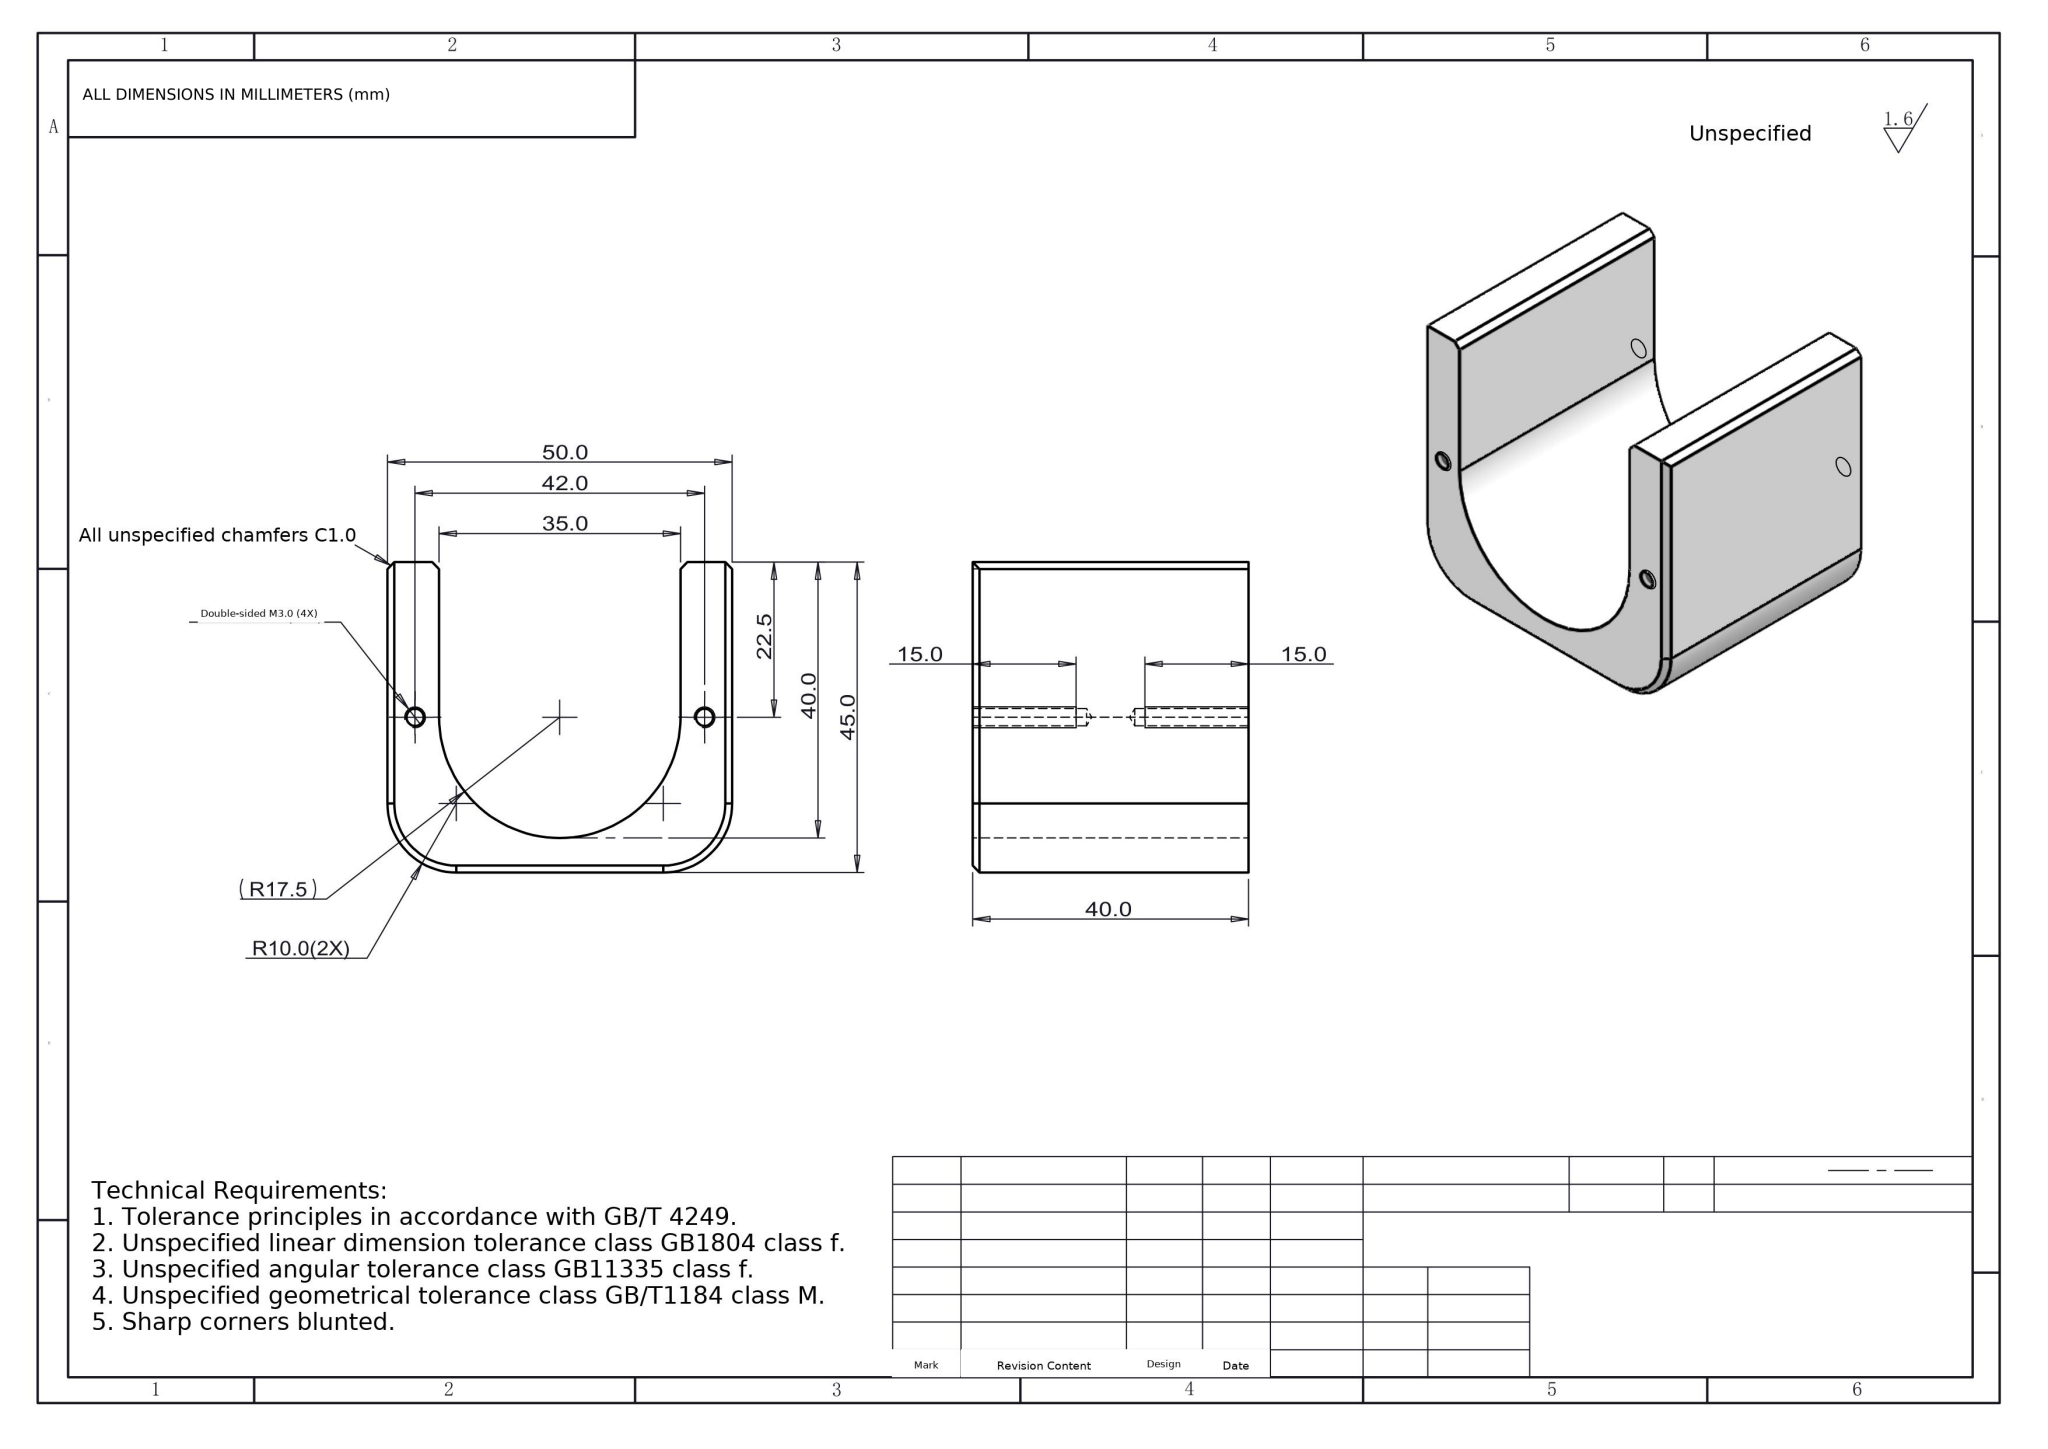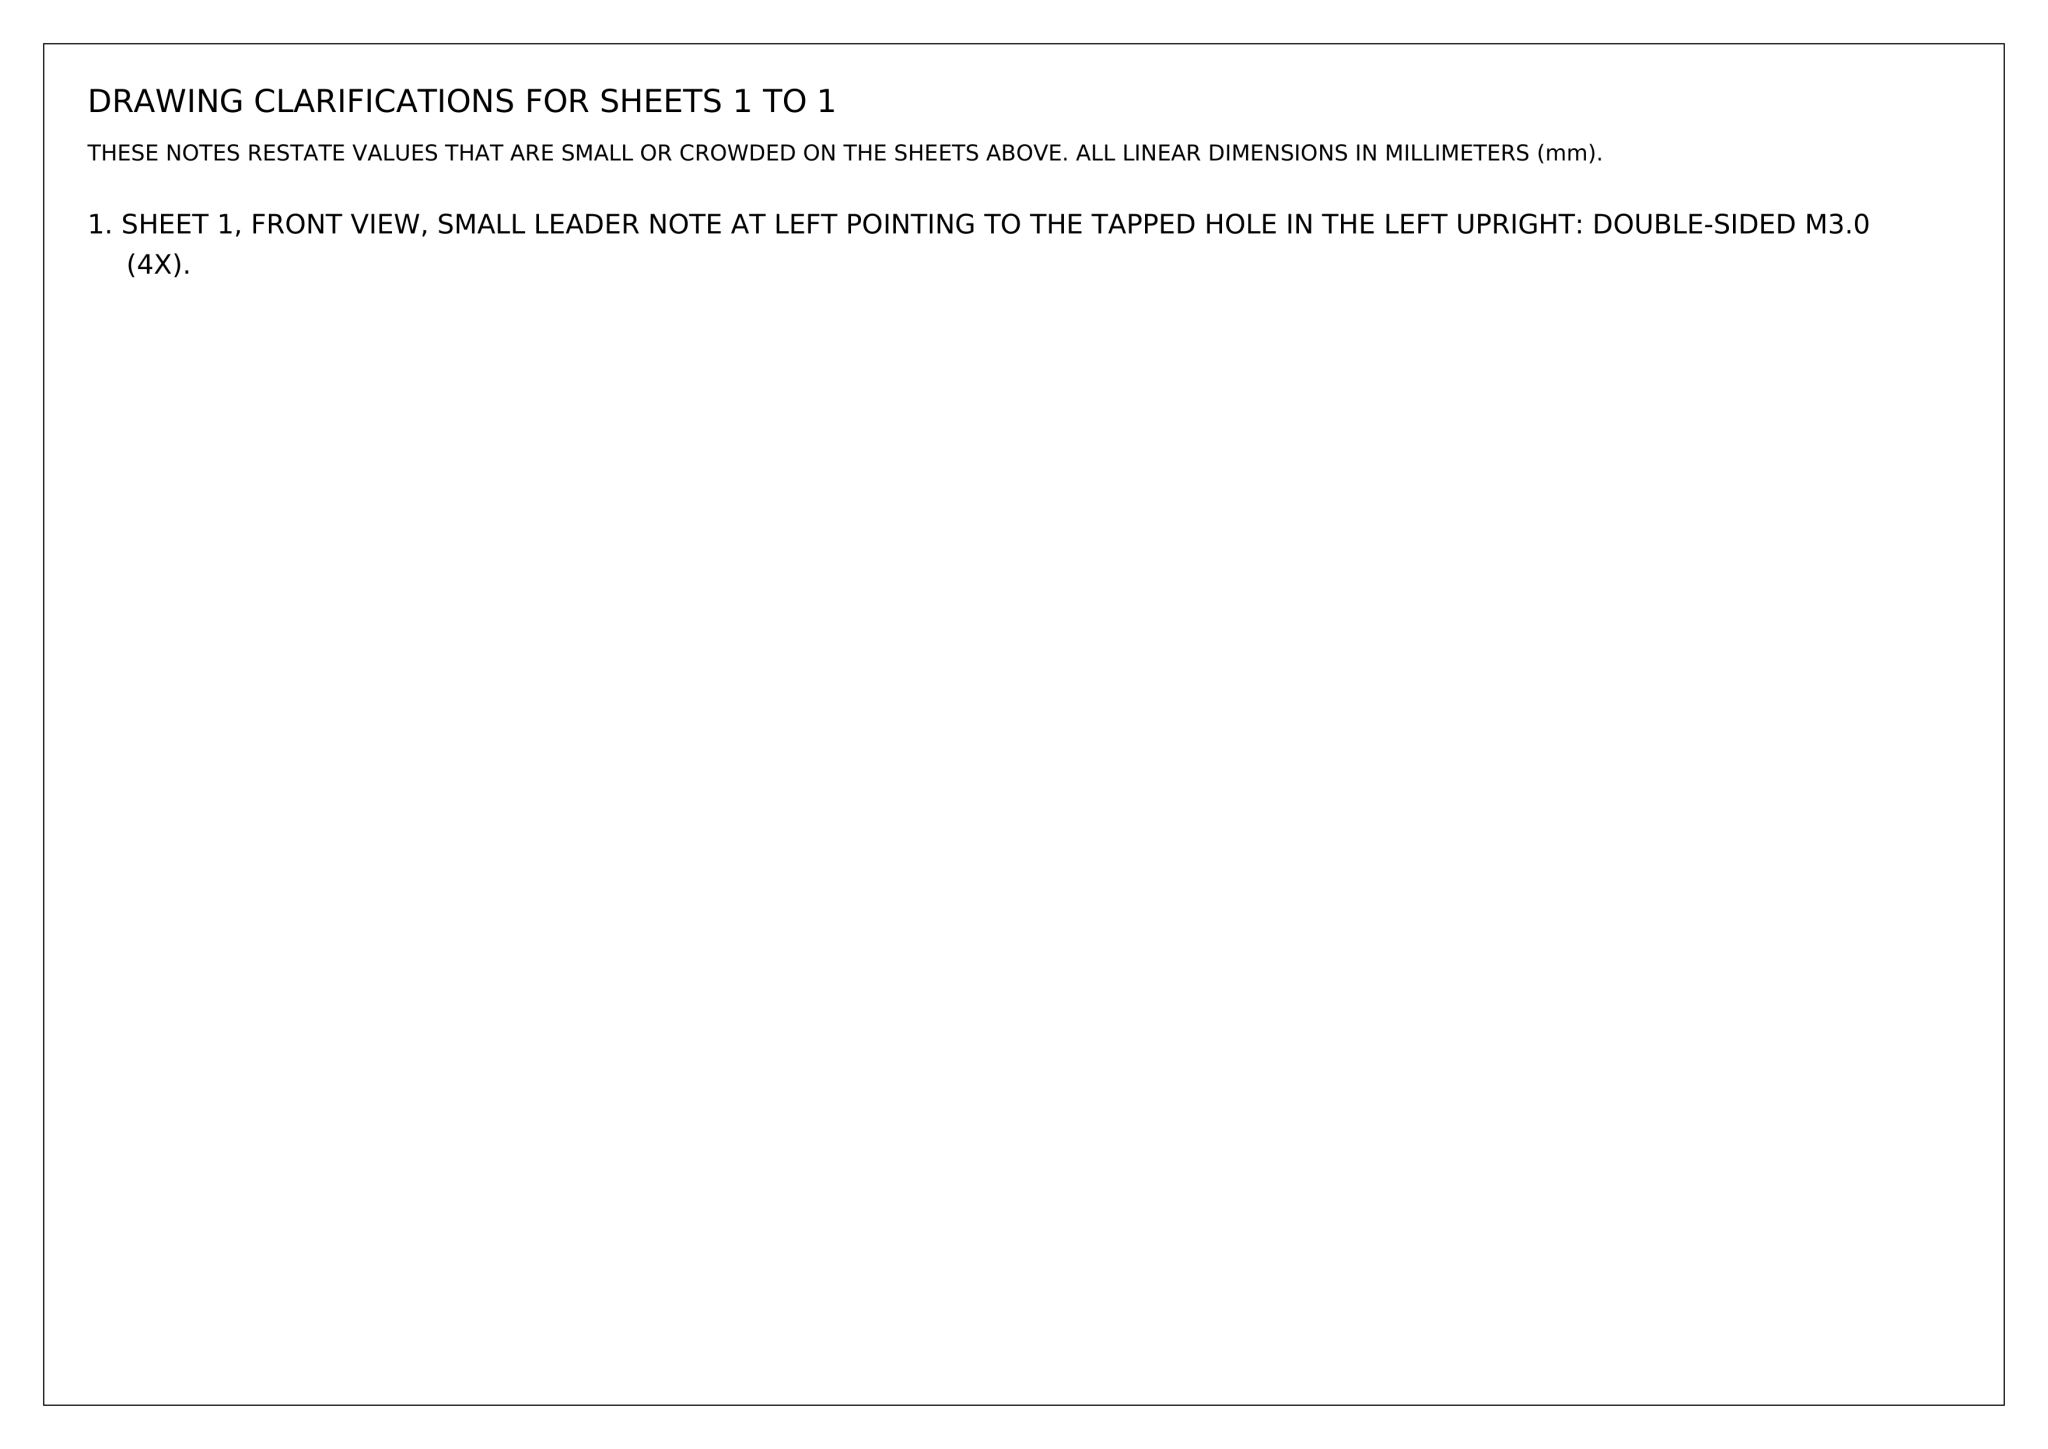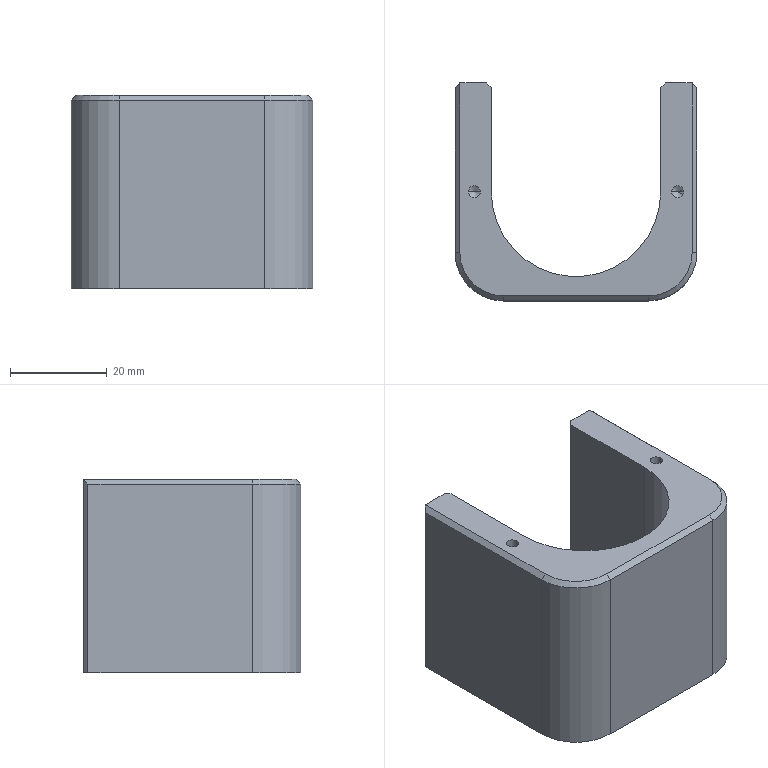Part | NX | mm | 1 solid | 37 faces | box 50 x 45 x 40 mm | volume 37068 mm3 | plane 16 | cylinder 11 | cone 10 | commonest cylinder face diameters 2.5 x8 20 x2 35 x1